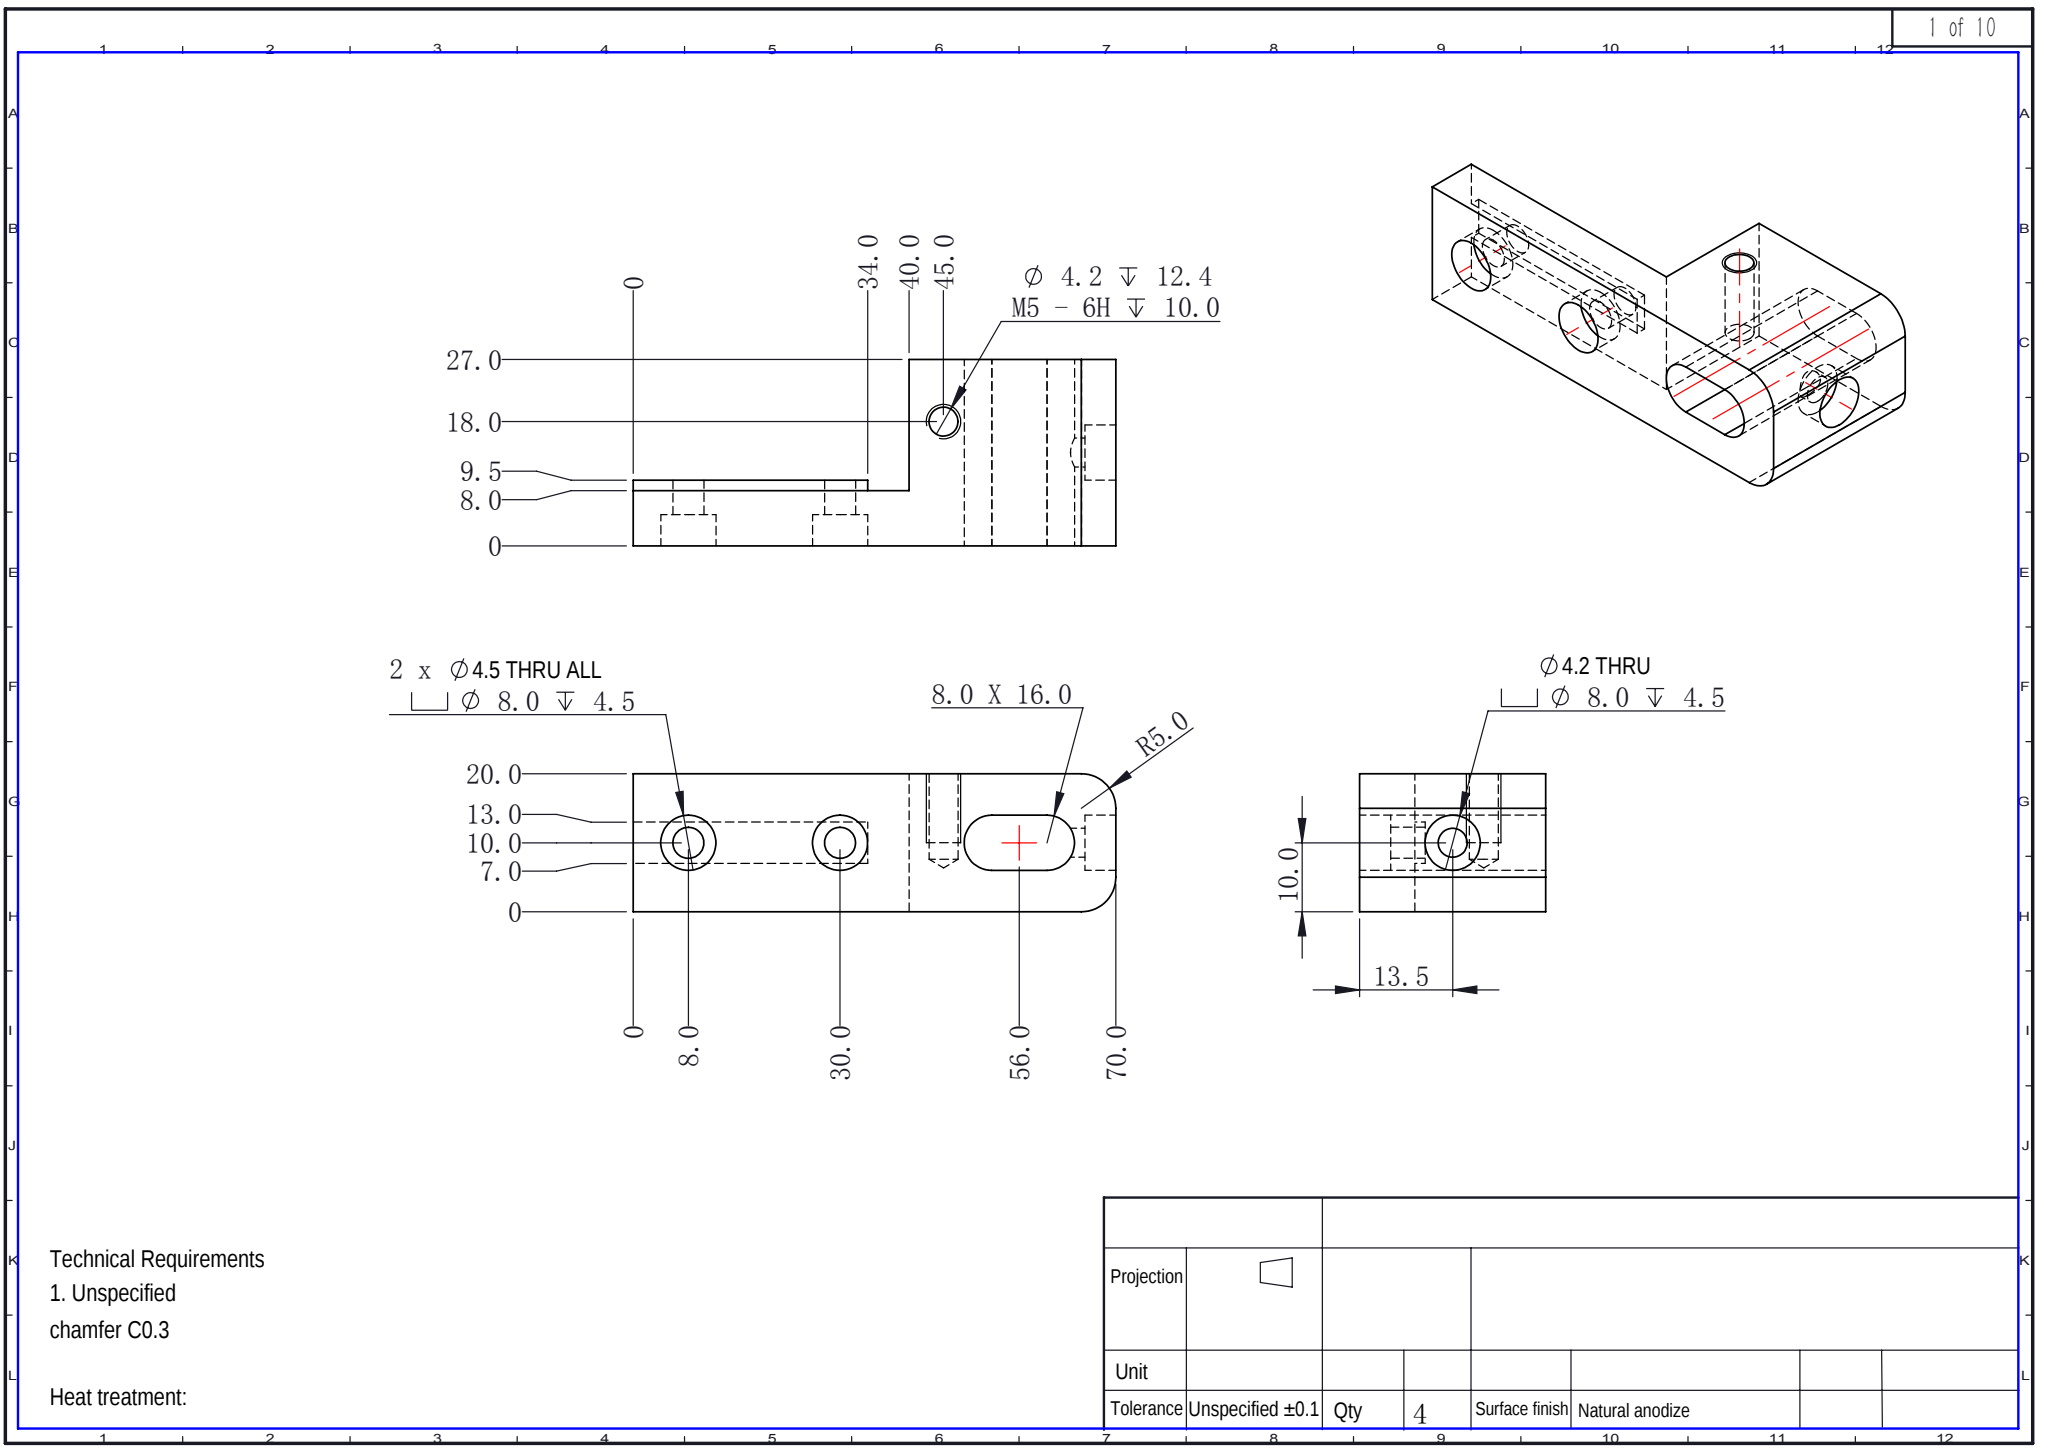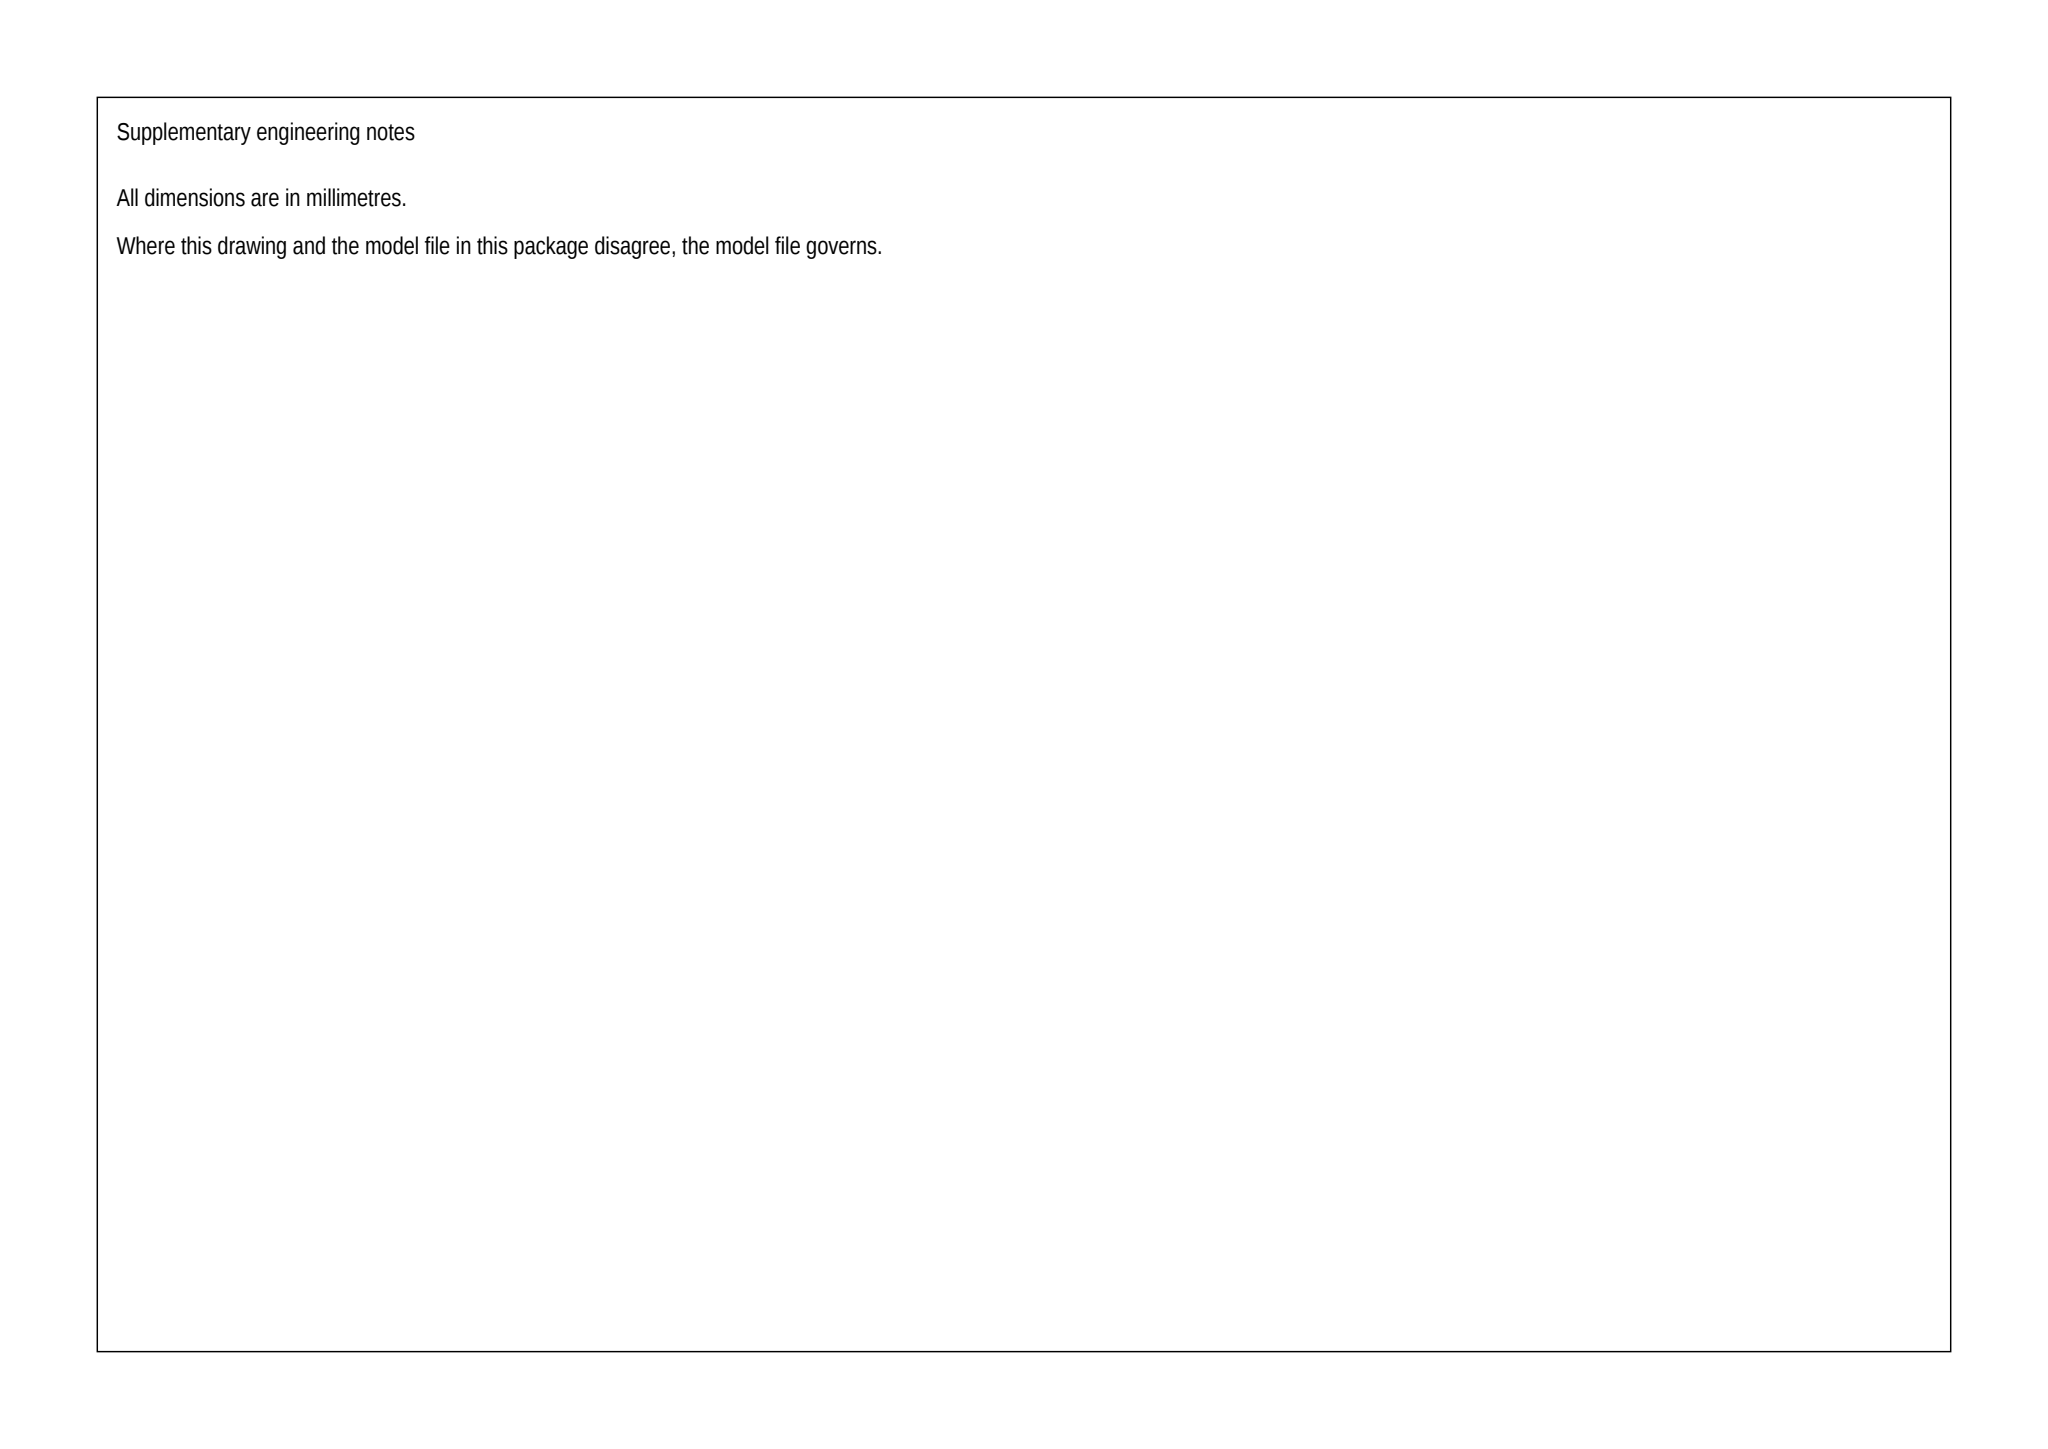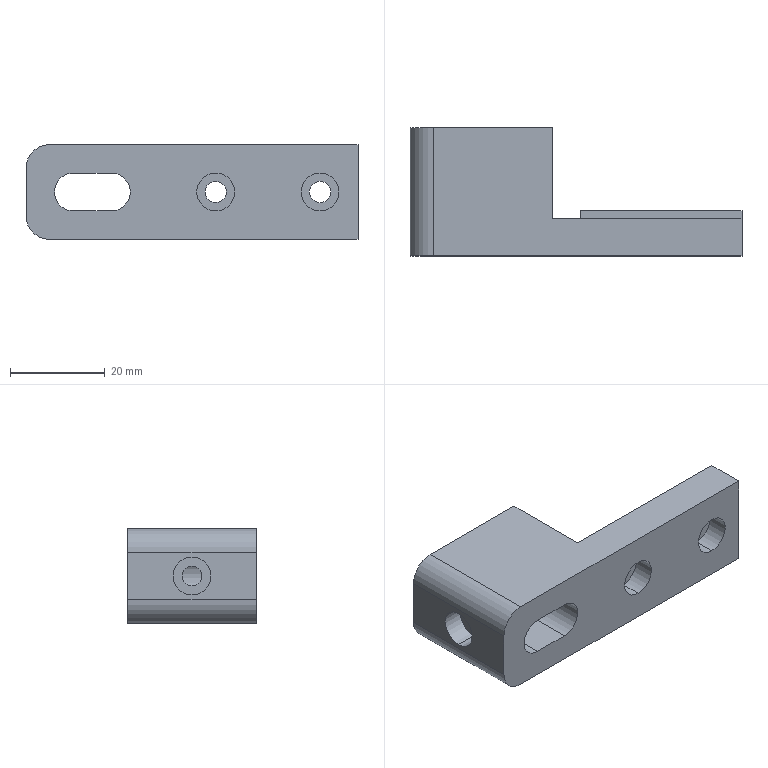Part | SolidWorks | mm | 1 solid | 37 faces | box 70 x 27 x 20 mm | volume 18493 mm3 | cylinder 18 | plane 17 | cone 2 | commonest cylinder face diameters 8 x8 4.2 x4 4.5 x4 10 x2